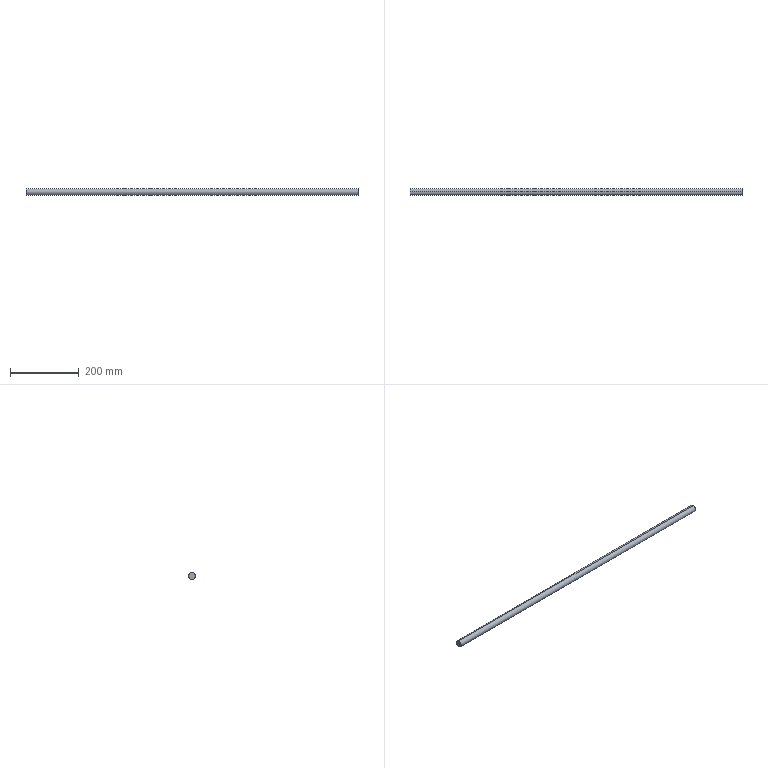Component | SolidWorks | DC-Motor-114-2 | 1 solid | 4 faces | box 965 x 20 x 20 mm | volume 303164 mm3 | cylinder 2 | plane 2 | commonest cylinder face diameters 20 x2
build123d program:
from build123d import *

# Parameters (mm, degrees)
SKETCH1_R           = 10
BOSS_EXTRUDE1_DEPTH = 482.5


with BuildPart() as part:
    # Sketch1 → Boss-Extrude1 (new, symmetric)
    with BuildSketch(Plane(origin=(0, 0, 0), x_dir=(0, 0, -1), z_dir=(1, 0, 0))):
        Circle(SKETCH1_R)
    extrude(amount=BOSS_EXTRUDE1_DEPTH, both=True)


solid = part.part

# Placed as in the assembly
solid = solid.moved(Location((3.208, -173.199, -389), (0, 0, 0)))
STEP:
#1=COLOUR_RGB('',0.7922,0.8196,0.9333);
#2=FILL_AREA_STYLE_COLOUR('',#1);
#3=FILL_AREA_STYLE('',(#2));
#4=SURFACE_STYLE_FILL_AREA(#3);
#5=SURFACE_SIDE_STYLE('',(#4));
#6=SURFACE_STYLE_USAGE(.BOTH.,#5);
#7=PRESENTATION_STYLE_ASSIGNMENT((#6));
#8=CARTESIAN_POINT('',(19.122,-6.819,-14.921));
#9=VERTEX_POINT('',#8);
#10=CARTESIAN_POINT('',(19.122,-6.819,-15.709));
#11=VERTEX_POINT('',#10);
#12=CARTESIAN_POINT('',(19.122,-6.819,-15.315));
#13=DIRECTION('',(1.,0.,0.));
#14=DIRECTION('',(0.,0.,1.));
#15=AXIS2_PLACEMENT_3D('',#12,#13,#14);
#16=CIRCLE('',#15,0.3937);
#17=EDGE_CURVE('',#9,#11,#16,.T.);
#18=ORIENTED_EDGE('',*,*,#17,.F.);
#19=CARTESIAN_POINT('',(-18.87,-6.819,-14.921));
#20=VERTEX_POINT('',#19);
#21=CARTESIAN_POINT('',(19.122,-6.819,-14.921));
#22=DIRECTION('',(-1.,-0.,-0.));
#23=VECTOR('',#22,39.37);
#24=LINE('',#21,#23);
#25=EDGE_CURVE('',#9,#20,#24,.T.);
#26=ORIENTED_EDGE('',*,*,#25,.T.);
#27=CARTESIAN_POINT('',(-18.87,-6.819,-15.709));
#28=VERTEX_POINT('',#27);
#29=CARTESIAN_POINT('',(-18.87,-6.819,-15.315));
#30=DIRECTION('',(1.,0.,0.));
#31=DIRECTION('',(0.,0.,1.));
#32=AXIS2_PLACEMENT_3D('',#29,#30,#31);
#33=CIRCLE('',#32,0.3937);
#34=EDGE_CURVE('',#20,#28,#33,.T.);
#35=ORIENTED_EDGE('',*,*,#34,.T.);
#36=CARTESIAN_POINT('',(19.122,-6.819,-15.709));
#37=DIRECTION('',(-1.,-0.,-0.));
#38=VECTOR('',#37,39.37);
#39=LINE('',#36,#38);
#40=EDGE_CURVE('',#11,#28,#39,.T.);
#41=ORIENTED_EDGE('',*,*,#40,.F.);
#42=EDGE_LOOP('',(#18,#26,#35,#41));
#43=FACE_OUTER_BOUND('',#42,.T.);
#44=CARTESIAN_POINT('',(19.122,-6.819,-15.315));
#45=DIRECTION('',(-1.,-0.,-0.));
#46=DIRECTION('',(0.,0.,-1.));
#47=AXIS2_PLACEMENT_3D('',#44,#45,#46);
#48=CYLINDRICAL_SURFACE('',#47,0.3937);
#49=ADVANCED_FACE('',(#43),#48,.T.);
#50=ORIENTED_EDGE('',*,*,#25,.F.);
#51=CARTESIAN_POINT('',(19.122,-6.819,-15.315));
#52=DIRECTION('',(1.,0.,0.));
#53=DIRECTION('',(0.,0.,1.));
#54=AXIS2_PLACEMENT_3D('',#51,#52,#53);
#55=CIRCLE('',#54,0.3937);
#56=EDGE_CURVE('',#11,#9,#55,.T.);
#57=ORIENTED_EDGE('',*,*,#56,.F.);
#58=ORIENTED_EDGE('',*,*,#40,.T.);
#59=CARTESIAN_POINT('',(-18.87,-6.819,-15.315));
#60=DIRECTION('',(1.,0.,0.));
#61=DIRECTION('',(0.,0.,1.));
#62=AXIS2_PLACEMENT_3D('',#59,#60,#61);
#63=CIRCLE('',#62,0.3937);
#64=EDGE_CURVE('',#28,#20,#63,.T.);
#65=ORIENTED_EDGE('',*,*,#64,.T.);
#66=EDGE_LOOP('',(#50,#57,#58,#65));
#67=FACE_OUTER_BOUND('',#66,.T.);
#68=CARTESIAN_POINT('',(19.122,-6.819,-15.315));
#69=DIRECTION('',(-1.,-0.,-0.));
#70=DIRECTION('',(0.,0.,-1.));
#71=AXIS2_PLACEMENT_3D('',#68,#69,#70);
#72=CYLINDRICAL_SURFACE('',#71,0.3937);
#73=ADVANCED_FACE('',(#67),#72,.T.);
#74=ORIENTED_EDGE('',*,*,#56,.T.);
#75=ORIENTED_EDGE('',*,*,#17,.T.);
#76=EDGE_LOOP('',(#74,#75));
#77=FACE_OUTER_BOUND('',#76,.T.);
#78=CARTESIAN_POINT('',(19.122,-6.819,-15.315));
#79=DIRECTION('',(1.,0.,0.));
#80=DIRECTION('',(0.,-0.,1.));
#81=AXIS2_PLACEMENT_3D('',#78,#79,#80);
#82=PLANE('',#81);
#83=ADVANCED_FACE('',(#77),#82,.T.);
#84=ORIENTED_EDGE('',*,*,#64,.F.);
#85=ORIENTED_EDGE('',*,*,#34,.F.);
#86=EDGE_LOOP('',(#84,#85));
#87=FACE_OUTER_BOUND('',#86,.T.);
#88=CARTESIAN_POINT('',(-18.87,-6.819,-15.315));
#89=DIRECTION('',(1.,0.,0.));
#90=DIRECTION('',(0.,-0.,1.));
#91=AXIS2_PLACEMENT_3D('',#88,#89,#90);
#92=PLANE('',#91);
#93=ADVANCED_FACE('',(#87),#92,.F.);
#94=CLOSED_SHELL('',(#49,#73,#83,#93));
#95=MANIFOLD_SOLID_BREP('',#94);
#96=STYLED_ITEM('',(#7),#95);
#97=(LENGTH_UNIT()NAMED_UNIT(*)SI_UNIT($,.METRE.));
#98=LENGTH_MEASURE_WITH_UNIT(LENGTH_MEASURE(0.0254),#97);
#99=DIMENSIONAL_EXPONENTS(1.,0.,0.,0.,0.,0.,0.);
#100=(CONVERSION_BASED_UNIT('',#98)LENGTH_UNIT()NAMED_UNIT(#99));
#101=UNCERTAINTY_MEASURE_WITH_UNIT(LENGTH_MEASURE(0.00001),#100,'','');
#102=(NAMED_UNIT(*)PLANE_ANGLE_UNIT()SI_UNIT($,.RADIAN.));
#103=(NAMED_UNIT(*)SI_UNIT($,.STERADIAN.)SOLID_ANGLE_UNIT());
#104=(GEOMETRIC_REPRESENTATION_CONTEXT(3)GLOBAL_UNCERTAINTY_ASSIGNED_CONTEXT((#101))GLOBAL_UNIT_ASSIGNED_CONTEXT((#100,#102,#103))REPRESENTATION_CONTEXT('',''));
#105=MECHANICAL_DESIGN_GEOMETRIC_PRESENTATION_REPRESENTATION('',(#96),#104);
#106=CARTESIAN_POINT('',(0.,0.,0.));
#107=DIRECTION('',(0.,0.,1.));
#108=DIRECTION('',(1.,0.,0.));
#109=AXIS2_PLACEMENT_3D('',#106,#107,#108);
#110=(LENGTH_UNIT()NAMED_UNIT(*)SI_UNIT($,.METRE.));
#111=LENGTH_MEASURE_WITH_UNIT(LENGTH_MEASURE(0.0254),#110);
#112=DIMENSIONAL_EXPONENTS(1.,0.,0.,0.,0.,0.,0.);
#113=(CONVERSION_BASED_UNIT('',#111)LENGTH_UNIT()NAMED_UNIT(#112));
#114=UNCERTAINTY_MEASURE_WITH_UNIT(LENGTH_MEASURE(0.00001),#113,'','');
#115=(NAMED_UNIT(*)PLANE_ANGLE_UNIT()SI_UNIT($,.RADIAN.));
#116=(NAMED_UNIT(*)SI_UNIT($,.STERADIAN.)SOLID_ANGLE_UNIT());
#117=(GEOMETRIC_REPRESENTATION_CONTEXT(3)GLOBAL_UNCERTAINTY_ASSIGNED_CONTEXT((#114))GLOBAL_UNIT_ASSIGNED_CONTEXT((#113,#115,#116))REPRESENTATION_CONTEXT('',''));
#118=ADVANCED_BREP_SHAPE_REPRESENTATION('',(#95,#109),#117);
#119=PRESENTATION_LAYER_ASSIGNMENT('','',(#96));